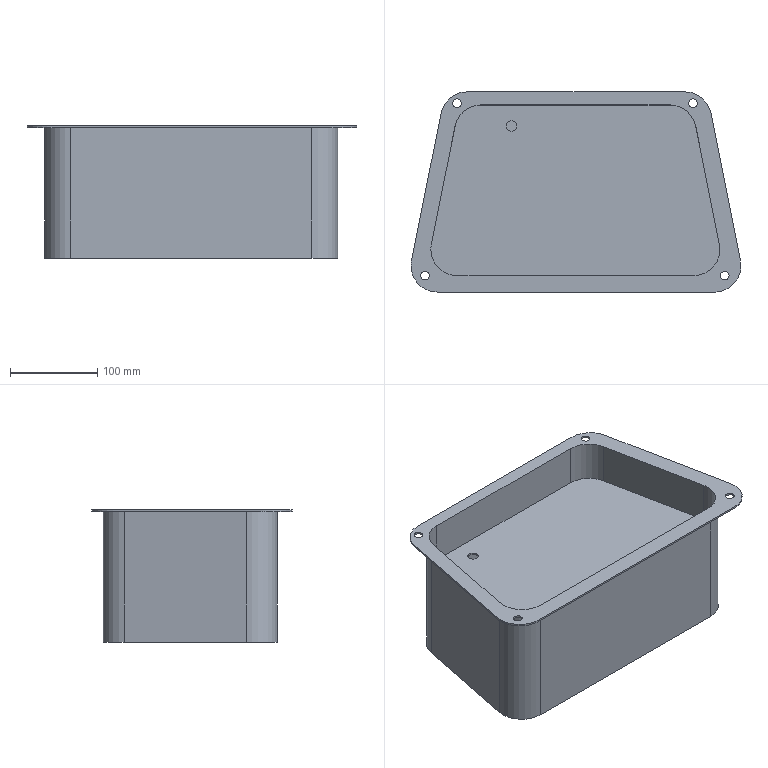Component | SolidWorks | DriveGuard-1 | 1 solid | 60 faces | box 378.81 x 230 x 152 mm | volume 529525 mm3 | cylinder 34 | plane 26 | commonest cylinder face diameters 60 x24 10 x8 12 x2
build123d program:
from build123d import *

# Parameters (mm, degrees)
BOSS_EXTRUDE1_DEPTH              = 150
SHELL1_T                         = -2
BOSS_EXTRUDE2_DEPTH              = 2
FILLET1_R                        = 30
SKETCH3_R                        = 5
CUT_EXTRUDE1_DEPTH               = 10
BOSS_EXTRUDE3_DEPTH              = 2
SKETCH5_W                        = 220
SKETCH5_H                        = 120
CUT_EXTRUDE2_DEPTH               = 2
FILLET2_R                        = 30
SKETCH1_R                        = 6
REPAIR_MOTORSHAFTCLEARANCE_DEPTH = 3


with BuildPart() as part:
    # Sketch1_2 → Boss-Extrude1 (new body)
    with BuildSketch(Plane(origin=(0, 0, 0), x_dir=(0, 0, -1), z_dir=(1, 0, 0))):
        Polygon((0, 0), (270, 0), (310, -200), (-40, -200), align=None)
    extrude(amount=BOSS_EXTRUDE1_DEPTH)

    # Shell1
    shell1_openings = [part.faces().sort_by_distance(p)[0] for p in [
        (0, -104.301, -135),
    ]]
    offset(amount=SHELL1_T, openings=shell1_openings, kind=Kind.INTERSECTION)

    # Sketch2 → Boss-Extrude2 (add)
    with BuildSketch(Plane.ZY):
        Polygon((-284.244, 13), (15.756, 13), (61.756, -217), (-330.244, -217), align=None)
        Polygon((-268.36, -2), (-1.64, -2), (37.56, -198), (-307.56, -198), align=None, mode=Mode.SUBTRACT)
    extrude(amount=BOSS_EXTRUDE2_DEPTH)

    # Fillet1
    fillet1_edges = [part.edges().sort_by_distance(p)[0] for p in [
        (73, -2, -1.64),
        (73, -198, 37.56),
        (73, -198, -307.56),
        (73, -2, -268.36),
        (-1, 13, -284.244),
        (-1, -217, -330.244),
        (-1, -217, 61.756),
        (-1, 13, 15.756),
        (75, 0, 0),
        (75, 0, -270),
        (75, -200, -310),
        (75, -200, 40),
    ]]
    fillet(fillet1_edges, radius=FILLET1_R)

    # Sketch3 → Cut-Extrude1 (cut)
    with BuildSketch(Plane(origin=(0, 0, 0), x_dir=(0, 0, -1), z_dir=(1, 0, 0))):
        Circle(SKETCH3_R)
        with Locations((270.93, 0)):
            Circle(SKETCH3_R)
        with Locations((-36.566, -198.045)):
            Circle(SKETCH3_R)
        with Locations((307.737, -198.045)):
            Circle(SKETCH3_R)
    extrude(amount=-CUT_EXTRUDE1_DEPTH, mode=Mode.SUBTRACT)

    # Sketch4 → Boss-Extrude3 (add)
    with BuildSketch(Plane.ZY.offset(-48)):
        with BuildLine():
            Line((-25.188, 0), (-245.406, 0))
            ThreePointArc((-245.406, 0), (-264.426, -6.8), (-274.823, -24.117))
            Line((-274.823, -24.117), (-302.823, -164.117))
            ThreePointArc((-302.823, -164.117), (-296.606, -189.02), (-273.406, -200))
            Line((-273.406, -200), (2.812, -200))
            ThreePointArc((2.812, -200), (26.012, -189.02), (32.229, -164.117))
            Line((32.229, -164.117), (4.229, -24.117))
            ThreePointArc((4.229, -24.117), (-6.169, -6.8), (-25.188, 0))
        make_face()
    extrude(amount=BOSS_EXTRUDE3_DEPTH)

    # Sketch5 → Cut-Extrude2 (cut)
    with BuildSketch(Plane(origin=(150, 0, 0), x_dir=(0, 0, -1), z_dir=(1, 0, 0))):
        with Locations((132.42, -100)):
            Rectangle(SKETCH5_W, SKETCH5_H)
    extrude(amount=-CUT_EXTRUDE2_DEPTH, mode=Mode.SUBTRACT)

    # Fillet2
    fillet2_edges = [part.edges().sort_by_distance(p)[0] for p in [
        (149, -40, -242.42),
        (149, -160, -242.42),
        (149, -160, -22.42),
        (149, -40, -22.42),
    ]]
    fillet(fillet2_edges, radius=FILLET2_R)

    # Sketch1 → Repair_MotorShaftClearance (cut, symmetric)
    with BuildSketch(Plane.ZY.offset(-46)):
        with Locations(Location((-208.467, -26, 0), (0, 0, 180))):
            Circle(SKETCH1_R)
    extrude(amount=REPAIR_MOTORSHAFTCLEARANCE_DEPTH, both=True, mode=Mode.SUBTRACT)


solid = part.part

# Placed as in the assembly
solid = solid.moved(Location((454.708, -241.715, 1459.724), (0, 90, 0)))